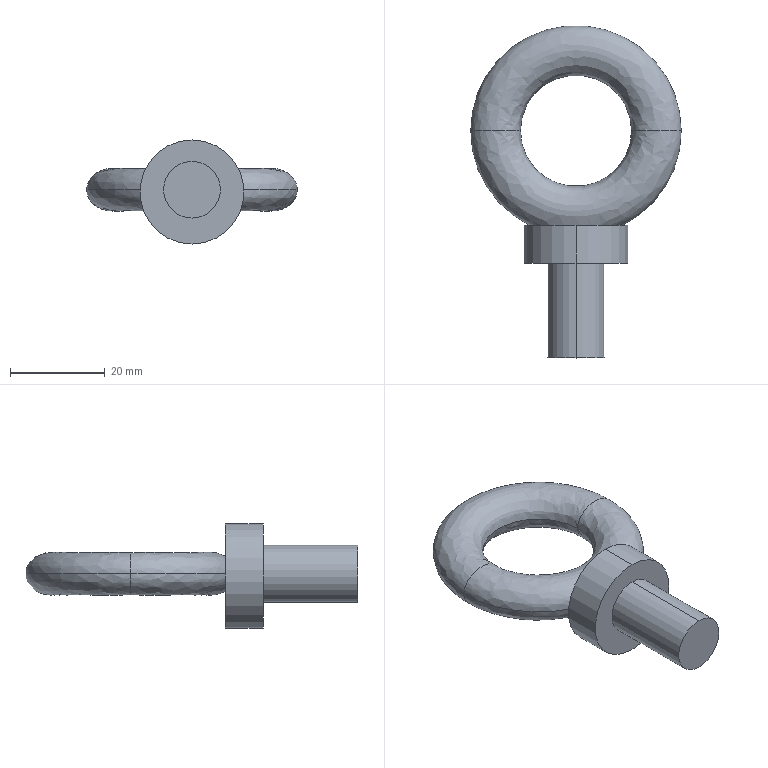Component | SolidWorks | M12LiftingEye-1 | 1 solid | 11 faces | box 44.49 x 70.25 x 22 mm | volume 13093 mm3 | spline 4 | cylinder 4 | plane 3 | commonest cylinder face diameters 12 x2 22 x2
build123d program:
from build123d import *

# Parameters (mm, degrees)
SKETCH2_RX          = 5.25
SKETCH2_RY          = 4.5
SKETCH3_R           = 11
BOSS_EXTRUDE1_DEPTH = 8
SKETCH4_R           = 6
BOSS_EXTRUDE2_DEPTH = 20


with BuildPart() as part:
    # Sweep1: sweep along a path in Sketch1
    with BuildLine(Plane.XY) as sweep1_path:
        CenterArc((0, 0), 17, 0, 360)
    # Sketch2 → Sweep1 (sweep)
    with BuildSketch(Plane(origin=(0, 0, 0), x_dir=(1, 0, 0), z_dir=(0, 1, 0))):
        with Locations(Location((16.996, 0), (0, 0, 180))):
            Ellipse(SKETCH2_RX, SKETCH2_RY)
    sweep(path=sweep1_path.line)

    # Sketch3 → Boss-Extrude1 (add)
    with BuildSketch(Plane(origin=(0, -20, 0), x_dir=(1, 0, 0), z_dir=(0, 1, 0))):
        with Locations(Location((0, 0.4774, 0), (0, 0, 270))):
            Circle(SKETCH3_R)
    extrude(amount=-BOSS_EXTRUDE1_DEPTH)

    # Sketch4 → Boss-Extrude2 (add)
    with BuildSketch(Plane.XZ.offset(28)):
        with Locations(Location((0, 0, 0), (0, 0, 90))):
            Circle(SKETCH4_R)
    extrude(amount=BOSS_EXTRUDE2_DEPTH)


solid = part.part

# Placed as in the assembly
solid = solid.moved(Location((347.082, 921.072, 1378.206), (0, 0, 0)))
STEP:
#1=COLOUR_RGB('',0.7922,0.8196,0.9333);
#2=FILL_AREA_STYLE_COLOUR('',#1);
#3=FILL_AREA_STYLE('',(#2));
#4=SURFACE_STYLE_FILL_AREA(#3);
#5=SURFACE_SIDE_STYLE('',(#4));
#6=SURFACE_STYLE_USAGE(.BOTH.,#5);
#7=PRESENTATION_STYLE_ASSIGNMENT((#6));
#8=CARTESIAN_POINT('',(14.127,36.263,54.26));
#9=VERTEX_POINT('',#8);
#10=CARTESIAN_POINT('',(13.202,36.263,54.26));
#11=VERTEX_POINT('',#10);
#12=CARTESIAN_POINT('',(13.665,36.263,54.26));
#13=DIRECTION('',(0.,0.,-1.));
#14=DIRECTION('',(1.,0.,0.));
#15=AXIS2_PLACEMENT_3D('',#12,#13,#14);
#16=CIRCLE('',#15,0.4624);
#17=EDGE_CURVE('',#9,#11,#16,.T.);
#18=ORIENTED_EDGE('',*,*,#17,.T.);
#19=CARTESIAN_POINT('',(12.789,36.263,54.26));
#20=VERTEX_POINT('',#19);
#21=CARTESIAN_POINT('',(13.202,36.263,54.26));
#22=CARTESIAN_POINT('',(13.202,36.263,54.614));
#23=CARTESIAN_POINT('',(12.789,36.263,54.614));
#24=CARTESIAN_POINT('',(12.789,36.263,54.26));
#25=(BOUNDED_CURVE()B_SPLINE_CURVE(3,(#21,#22,#23,#24),.UNSPECIFIED.,.F.,.T.)B_SPLINE_CURVE_WITH_KNOTS((4,4),(0.,3.142),.UNSPECIFIED.)CURVE()GEOMETRIC_REPRESENTATION_ITEM()RATIONAL_B_SPLINE_CURVE((1.,0.3333,0.3333,1.))REPRESENTATION_ITEM(''));
#26=EDGE_CURVE('',#11,#20,#25,.T.);
#27=ORIENTED_EDGE('',*,*,#26,.T.);
#28=CARTESIAN_POINT('',(13.281,35.475,54.26));
#29=VERTEX_POINT('',#28);
#30=CARTESIAN_POINT('',(13.665,36.263,54.26));
#31=DIRECTION('',(0.,0.,-1.));
#32=DIRECTION('',(1.,0.,0.));
#33=AXIS2_PLACEMENT_3D('',#30,#31,#32);
#34=CIRCLE('',#33,0.8758);
#35=EDGE_CURVE('',#29,#20,#34,.T.);
#36=ORIENTED_EDGE('',*,*,#35,.F.);
#37=CARTESIAN_POINT('',(14.048,35.475,54.26));
#38=VERTEX_POINT('',#37);
#39=CARTESIAN_POINT('',(13.281,35.475,54.26));
#40=CARTESIAN_POINT('',(13.281,35.475,54.265));
#41=CARTESIAN_POINT('',(13.282,35.475,54.269));
#42=CARTESIAN_POINT('',(13.284,35.475,54.278));
#43=CARTESIAN_POINT('',(13.285,35.475,54.283));
#44=CARTESIAN_POINT('',(13.29,35.475,54.296));
#45=CARTESIAN_POINT('',(13.296,35.475,54.304));
#46=CARTESIAN_POINT('',(13.307,35.475,54.318));
#47=CARTESIAN_POINT('',(13.314,35.475,54.324));
#48=CARTESIAN_POINT('',(13.329,35.475,54.336));
#49=CARTESIAN_POINT('',(13.336,35.475,54.341));
#50=CARTESIAN_POINT('',(13.36,35.475,54.355));
#51=CARTESIAN_POINT('',(13.377,35.475,54.362));
#52=CARTESIAN_POINT('',(13.412,35.475,54.375));
#53=CARTESIAN_POINT('',(13.429,35.475,54.38));
#54=CARTESIAN_POINT('',(13.483,35.475,54.392));
#55=CARTESIAN_POINT('',(13.519,35.475,54.397));
#56=CARTESIAN_POINT('',(13.574,35.475,54.402));
#57=CARTESIAN_POINT('',(13.592,35.475,54.403));
#58=CARTESIAN_POINT('',(13.629,35.475,54.405));
#59=CARTESIAN_POINT('',(13.647,35.475,54.405));
#60=CARTESIAN_POINT('',(13.702,35.475,54.405));
#61=CARTESIAN_POINT('',(13.739,35.475,54.404));
#62=CARTESIAN_POINT('',(13.811,35.475,54.397));
#63=CARTESIAN_POINT('',(13.847,35.475,54.392));
#64=CARTESIAN_POINT('',(13.901,35.475,54.38));
#65=CARTESIAN_POINT('',(13.918,35.475,54.375));
#66=CARTESIAN_POINT('',(13.953,35.475,54.362));
#67=CARTESIAN_POINT('',(13.969,35.475,54.355));
#68=CARTESIAN_POINT('',(13.993,35.475,54.341));
#69=CARTESIAN_POINT('',(14.001,35.475,54.336));
#70=CARTESIAN_POINT('',(14.015,35.475,54.324));
#71=CARTESIAN_POINT('',(14.022,35.475,54.318));
#72=CARTESIAN_POINT('',(14.034,35.475,54.304));
#73=CARTESIAN_POINT('',(14.039,35.475,54.296));
#74=CARTESIAN_POINT('',(14.046,35.475,54.279));
#75=CARTESIAN_POINT('',(14.048,35.475,54.269));
#76=CARTESIAN_POINT('',(14.048,35.475,54.26));
#77=B_SPLINE_CURVE_WITH_KNOTS('',3,(#39,#40,#41,#42,#43,#44,#45,#46,#47,#48,#49,#50,#51,#52,#53,#54,#55,#56,#57,#58,#59,#60,#61,#62,#63,#64,#65,#66,#67,#68,#69,#70,#71,#72,#73,#74,#75,#76),.UNSPECIFIED.,.F.,.F.,(4,2,2,2,2,2,2,2,2,2,2,2,2,2,2,2,2,2,4),(0.03335,0.03369,0.03404,0.03473,0.03543,0.03612,0.03751,0.03889,0.04167,0.04305,0.04444,0.04721,0.04999,0.05138,0.05276,0.05346,0.05415,0.05484,0.05554),.UNSPECIFIED.);
#78=EDGE_CURVE('',#29,#38,#77,.T.);
#79=ORIENTED_EDGE('',*,*,#78,.T.);
#80=CARTESIAN_POINT('',(14.54,36.263,54.26));
#81=VERTEX_POINT('',#80);
#82=CARTESIAN_POINT('',(13.665,36.263,54.26));
#83=DIRECTION('',(0.,0.,-1.));
#84=DIRECTION('',(1.,0.,0.));
#85=AXIS2_PLACEMENT_3D('',#82,#83,#84);
#86=CIRCLE('',#85,0.8758);
#87=EDGE_CURVE('',#81,#38,#86,.T.);
#88=ORIENTED_EDGE('',*,*,#87,.F.);
#89=CARTESIAN_POINT('',(14.127,36.263,54.26));
#90=CARTESIAN_POINT('',(14.127,36.263,54.614));
#91=CARTESIAN_POINT('',(14.54,36.263,54.614));
#92=CARTESIAN_POINT('',(14.54,36.263,54.26));
#93=(BOUNDED_CURVE()B_SPLINE_CURVE(3,(#89,#90,#91,#92),.UNSPECIFIED.,.F.,.T.)B_SPLINE_CURVE_WITH_KNOTS((4,4),(0.,3.142),.UNSPECIFIED.)CURVE()GEOMETRIC_REPRESENTATION_ITEM()RATIONAL_B_SPLINE_CURVE((1.,0.3333,0.3333,1.))REPRESENTATION_ITEM(''));
#94=EDGE_CURVE('',#9,#81,#93,.T.);
#95=ORIENTED_EDGE('',*,*,#94,.F.);
#96=EDGE_LOOP('',(#18,#27,#36,#79,#88,#95));
#97=FACE_OUTER_BOUND('',#96,.T.);
#98=CARTESIAN_POINT('',(14.127,36.263,54.26));
#99=CARTESIAN_POINT('',(14.127,35.338,54.26));
#100=CARTESIAN_POINT('',(13.202,35.338,54.26));
#101=CARTESIAN_POINT('',(13.202,36.263,54.26));
#102=CARTESIAN_POINT('',(14.127,36.263,54.614));
#103=CARTESIAN_POINT('',(14.127,35.338,54.614));
#104=CARTESIAN_POINT('',(13.202,35.338,54.614));
#105=CARTESIAN_POINT('',(13.202,36.263,54.614));
#106=CARTESIAN_POINT('',(14.54,36.263,54.614));
#107=CARTESIAN_POINT('',(14.54,34.511,54.614));
#108=CARTESIAN_POINT('',(12.789,34.511,54.614));
#109=CARTESIAN_POINT('',(12.789,36.263,54.614));
#110=CARTESIAN_POINT('',(14.54,36.263,54.26));
#111=CARTESIAN_POINT('',(14.54,34.511,54.26));
#112=CARTESIAN_POINT('',(12.789,34.511,54.26));
#113=CARTESIAN_POINT('',(12.789,36.263,54.26));
#114=(BOUNDED_SURFACE()B_SPLINE_SURFACE(3,3,((#98,#99,#100,#101),(#102,#103,#104,#105),(#106,#107,#108,#109),(#110,#111,#112,#113)),.UNSPECIFIED.,.F.,.F.,.T.)B_SPLINE_SURFACE_WITH_KNOTS((4,4),(4,4),(0.,1.),(0.,1.),.UNSPECIFIED.)GEOMETRIC_REPRESENTATION_ITEM()RATIONAL_B_SPLINE_SURFACE(((1.,0.3333,0.3333,1.),(0.3333,0.1111,0.1111,0.3333),(0.3333,0.1111,0.1111,0.3333),(1.,0.3333,0.3333,1.)))REPRESENTATION_ITEM('')SURFACE());
#115=ADVANCED_FACE('',(#97),#114,.F.);
#116=ORIENTED_EDGE('',*,*,#35,.T.);
#117=CARTESIAN_POINT('',(12.789,36.263,54.26));
#118=CARTESIAN_POINT('',(12.789,36.263,53.906));
#119=CARTESIAN_POINT('',(13.202,36.263,53.906));
#120=CARTESIAN_POINT('',(13.202,36.263,54.26));
#121=(BOUNDED_CURVE()B_SPLINE_CURVE(3,(#117,#118,#119,#120),.UNSPECIFIED.,.F.,.T.)B_SPLINE_CURVE_WITH_KNOTS((4,4),(3.142,6.283),.UNSPECIFIED.)CURVE()GEOMETRIC_REPRESENTATION_ITEM()RATIONAL_B_SPLINE_CURVE((1.,0.3333,0.3333,1.))REPRESENTATION_ITEM(''));
#122=EDGE_CURVE('',#20,#11,#121,.T.);
#123=ORIENTED_EDGE('',*,*,#122,.T.);
#124=ORIENTED_EDGE('',*,*,#17,.F.);
#125=CARTESIAN_POINT('',(14.54,36.263,54.26));
#126=CARTESIAN_POINT('',(14.54,36.263,53.906));
#127=CARTESIAN_POINT('',(14.127,36.263,53.906));
#128=CARTESIAN_POINT('',(14.127,36.263,54.26));
#129=(BOUNDED_CURVE()B_SPLINE_CURVE(3,(#125,#126,#127,#128),.UNSPECIFIED.,.F.,.T.)B_SPLINE_CURVE_WITH_KNOTS((4,4),(3.142,6.283),.UNSPECIFIED.)CURVE()GEOMETRIC_REPRESENTATION_ITEM()RATIONAL_B_SPLINE_CURVE((1.,0.3333,0.3333,1.))REPRESENTATION_ITEM(''));
#130=EDGE_CURVE('',#81,#9,#129,.T.);
#131=ORIENTED_EDGE('',*,*,#130,.F.);
#132=ORIENTED_EDGE('',*,*,#87,.T.);
#133=CARTESIAN_POINT('',(14.048,35.475,54.26));
#134=CARTESIAN_POINT('',(14.048,35.475,54.255));
#135=CARTESIAN_POINT('',(14.048,35.475,54.251));
#136=CARTESIAN_POINT('',(14.046,35.475,54.242));
#137=CARTESIAN_POINT('',(14.044,35.475,54.237));
#138=CARTESIAN_POINT('',(14.039,35.475,54.224));
#139=CARTESIAN_POINT('',(14.034,35.475,54.217));
#140=CARTESIAN_POINT('',(14.022,35.475,54.202));
#141=CARTESIAN_POINT('',(14.015,35.475,54.196));
#142=CARTESIAN_POINT('',(14.001,35.475,54.184));
#143=CARTESIAN_POINT('',(13.993,35.475,54.179));
#144=CARTESIAN_POINT('',(13.969,35.475,54.165));
#145=CARTESIAN_POINT('',(13.952,35.475,54.158));
#146=CARTESIAN_POINT('',(13.918,35.475,54.145));
#147=CARTESIAN_POINT('',(13.9,35.475,54.14));
#148=CARTESIAN_POINT('',(13.847,35.475,54.128));
#149=CARTESIAN_POINT('',(13.811,35.475,54.123));
#150=CARTESIAN_POINT('',(13.738,35.475,54.116));
#151=CARTESIAN_POINT('',(13.701,35.475,54.115));
#152=CARTESIAN_POINT('',(13.628,35.475,54.115));
#153=CARTESIAN_POINT('',(13.592,35.475,54.116));
#154=CARTESIAN_POINT('',(13.519,35.475,54.123));
#155=CARTESIAN_POINT('',(13.483,35.475,54.128));
#156=CARTESIAN_POINT('',(13.429,35.475,54.14));
#157=CARTESIAN_POINT('',(13.411,35.475,54.145));
#158=CARTESIAN_POINT('',(13.377,35.475,54.158));
#159=CARTESIAN_POINT('',(13.36,35.475,54.165));
#160=CARTESIAN_POINT('',(13.337,35.475,54.179));
#161=CARTESIAN_POINT('',(13.329,35.475,54.184));
#162=CARTESIAN_POINT('',(13.314,35.475,54.196));
#163=CARTESIAN_POINT('',(13.307,35.475,54.202));
#164=CARTESIAN_POINT('',(13.295,35.475,54.216));
#165=CARTESIAN_POINT('',(13.29,35.475,54.224));
#166=CARTESIAN_POINT('',(13.285,35.475,54.237));
#167=CARTESIAN_POINT('',(13.284,35.475,54.242));
#168=CARTESIAN_POINT('',(13.282,35.475,54.251));
#169=CARTESIAN_POINT('',(13.281,35.475,54.255));
#170=CARTESIAN_POINT('',(13.281,35.475,54.26));
#171=B_SPLINE_CURVE_WITH_KNOTS('',3,(#133,#134,#135,#136,#137,#138,#139,#140,#141,#142,#143,#144,#145,#146,#147,#148,#149,#150,#151,#152,#153,#154,#155,#156,#157,#158,#159,#160,#161,#162,#163,#164,#165,#166,#167,#168,#169,#170),.UNSPECIFIED.,.F.,.F.,(4,2,2,2,2,2,2,2,2,2,2,2,2,2,2,2,2,2,4),(0.01112,0.01147,0.01181,0.01251,0.0132,0.0139,0.01529,0.01668,0.01945,0.02223,0.02501,0.02779,0.02918,0.03057,0.03126,0.03196,0.03265,0.033,0.03335),.UNSPECIFIED.);
#172=EDGE_CURVE('',#38,#29,#171,.T.);
#173=ORIENTED_EDGE('',*,*,#172,.T.);
#174=EDGE_LOOP('',(#116,#123,#124,#131,#132,#173));
#175=FACE_OUTER_BOUND('',#174,.T.);
#176=CARTESIAN_POINT('',(14.54,36.263,54.26));
#177=CARTESIAN_POINT('',(14.54,34.511,54.26));
#178=CARTESIAN_POINT('',(12.789,34.511,54.26));
#179=CARTESIAN_POINT('',(12.789,36.263,54.26));
#180=CARTESIAN_POINT('',(14.54,36.263,53.906));
#181=CARTESIAN_POINT('',(14.54,34.511,53.906));
#182=CARTESIAN_POINT('',(12.789,34.511,53.906));
#183=CARTESIAN_POINT('',(12.789,36.263,53.906));
#184=CARTESIAN_POINT('',(14.127,36.263,53.906));
#185=CARTESIAN_POINT('',(14.127,35.338,53.906));
#186=CARTESIAN_POINT('',(13.202,35.338,53.906));
#187=CARTESIAN_POINT('',(13.202,36.263,53.906));
#188=CARTESIAN_POINT('',(14.127,36.263,54.26));
#189=CARTESIAN_POINT('',(14.127,35.338,54.26));
#190=CARTESIAN_POINT('',(13.202,35.338,54.26));
#191=CARTESIAN_POINT('',(13.202,36.263,54.26));
#192=(BOUNDED_SURFACE()B_SPLINE_SURFACE(3,3,((#176,#177,#178,#179),(#180,#181,#182,#183),(#184,#185,#186,#187),(#188,#189,#190,#191)),.UNSPECIFIED.,.F.,.F.,.F.)B_SPLINE_SURFACE_WITH_KNOTS((4,4),(4,4),(0.,1.),(0.,1.),.UNSPECIFIED.)GEOMETRIC_REPRESENTATION_ITEM()RATIONAL_B_SPLINE_SURFACE(((1.,0.3333,0.3333,1.),(0.3333,0.1111,0.1111,0.3333),(0.3333,0.1111,0.1111,0.3333),(1.,0.3333,0.3333,1.)))REPRESENTATION_ITEM('')SURFACE());
#193=ADVANCED_FACE('',(#175),#192,.F.);
#194=CARTESIAN_POINT('',(13.665,34.373,54.024));
#195=VERTEX_POINT('',#194);
#196=CARTESIAN_POINT('',(13.665,34.373,54.496));
#197=VERTEX_POINT('',#196);
#198=CARTESIAN_POINT('',(13.665,34.373,54.26));
#199=DIRECTION('',(0.,-1.,0.));
#200=DIRECTION('',(0.,0.,-1.));
#201=AXIS2_PLACEMENT_3D('',#198,#199,#200);
#202=CIRCLE('',#201,0.2362);
#203=EDGE_CURVE('',#195,#197,#202,.T.);
#204=ORIENTED_EDGE('',*,*,#203,.F.);
#205=CARTESIAN_POINT('',(13.665,35.16,54.024));
#206=VERTEX_POINT('',#205);
#207=CARTESIAN_POINT('',(13.665,34.373,54.024));
#208=DIRECTION('',(0.,1.,0.));
#209=VECTOR('',#208,39.37);
#210=LINE('',#207,#209);
#211=EDGE_CURVE('',#195,#206,#210,.T.);
#212=ORIENTED_EDGE('',*,*,#211,.T.);
#213=CARTESIAN_POINT('',(13.665,35.16,54.496));
#214=VERTEX_POINT('',#213);
#215=CARTESIAN_POINT('',(13.665,35.16,54.26));
#216=DIRECTION('',(0.,-1.,0.));
#217=DIRECTION('',(0.,0.,1.));
#218=AXIS2_PLACEMENT_3D('',#215,#216,#217);
#219=CIRCLE('',#218,0.2362);
#220=EDGE_CURVE('',#206,#214,#219,.T.);
#221=ORIENTED_EDGE('',*,*,#220,.T.);
#222=CARTESIAN_POINT('',(13.665,34.373,54.496));
#223=DIRECTION('',(0.,1.,0.));
#224=VECTOR('',#223,39.37);
#225=LINE('',#222,#224);
#226=EDGE_CURVE('',#197,#214,#225,.T.);
#227=ORIENTED_EDGE('',*,*,#226,.F.);
#228=EDGE_LOOP('',(#204,#212,#221,#227));
#229=FACE_OUTER_BOUND('',#228,.T.);
#230=CARTESIAN_POINT('',(13.665,34.373,54.26));
#231=DIRECTION('',(0.,1.,0.));
#232=DIRECTION('',(0.,0.,1.));
#233=AXIS2_PLACEMENT_3D('',#230,#231,#232);
#234=CYLINDRICAL_SURFACE('',#233,0.2362);
#235=ADVANCED_FACE('',(#229),#234,.T.);
#236=ORIENTED_EDGE('',*,*,#122,.F.);
#237=CARTESIAN_POINT('',(13.665,36.263,54.26));
#238=DIRECTION('',(0.,0.,-1.));
#239=DIRECTION('',(1.,0.,0.));
#240=AXIS2_PLACEMENT_3D('',#237,#238,#239);
#241=CIRCLE('',#240,0.8758);
#242=EDGE_CURVE('',#20,#81,#241,.T.);
#243=ORIENTED_EDGE('',*,*,#242,.T.);
#244=ORIENTED_EDGE('',*,*,#130,.T.);
#245=CARTESIAN_POINT('',(13.665,36.263,54.26));
#246=DIRECTION('',(0.,0.,-1.));
#247=DIRECTION('',(1.,0.,0.));
#248=AXIS2_PLACEMENT_3D('',#245,#246,#247);
#249=CIRCLE('',#248,0.4624);
#250=EDGE_CURVE('',#11,#9,#249,.T.);
#251=ORIENTED_EDGE('',*,*,#250,.F.);
#252=EDGE_LOOP('',(#236,#243,#244,#251));
#253=FACE_OUTER_BOUND('',#252,.T.);
#254=CARTESIAN_POINT('',(12.789,36.263,54.26));
#255=CARTESIAN_POINT('',(12.789,38.014,54.26));
#256=CARTESIAN_POINT('',(14.54,38.014,54.26));
#257=CARTESIAN_POINT('',(14.54,36.263,54.26));
#258=CARTESIAN_POINT('',(12.789,36.263,53.906));
#259=CARTESIAN_POINT('',(12.789,38.014,53.906));
#260=CARTESIAN_POINT('',(14.54,38.014,53.906));
#261=CARTESIAN_POINT('',(14.54,36.263,53.906));
#262=CARTESIAN_POINT('',(13.202,36.263,53.906));
#263=CARTESIAN_POINT('',(13.202,37.188,53.906));
#264=CARTESIAN_POINT('',(14.127,37.188,53.906));
#265=CARTESIAN_POINT('',(14.127,36.263,53.906));
#266=CARTESIAN_POINT('',(13.202,36.263,54.26));
#267=CARTESIAN_POINT('',(13.202,37.188,54.26));
#268=CARTESIAN_POINT('',(14.127,37.188,54.26));
#269=CARTESIAN_POINT('',(14.127,36.263,54.26));
#270=(BOUNDED_SURFACE()B_SPLINE_SURFACE(3,3,((#254,#255,#256,#257),(#258,#259,#260,#261),(#262,#263,#264,#265),(#266,#267,#268,#269)),.UNSPECIFIED.,.F.,.F.,.T.)B_SPLINE_SURFACE_WITH_KNOTS((4,4),(4,4),(0.,1.),(0.,1.),.UNSPECIFIED.)GEOMETRIC_REPRESENTATION_ITEM()RATIONAL_B_SPLINE_SURFACE(((1.,0.3333,0.3333,1.),(0.3333,0.1111,0.1111,0.3333),(0.3333,0.1111,0.1111,0.3333),(1.,0.3333,0.3333,1.)))REPRESENTATION_ITEM('')SURFACE());
#271=ADVANCED_FACE('',(#253),#270,.F.);
#272=CARTESIAN_POINT('',(13.665,35.16,54.674));
#273=VERTEX_POINT('',#272);
#274=CARTESIAN_POINT('',(13.665,35.16,53.808));
#275=VERTEX_POINT('',#274);
#276=CARTESIAN_POINT('',(13.665,35.16,54.241));
#277=DIRECTION('',(0.,1.,0.));
#278=DIRECTION('',(0.,0.,1.));
#279=AXIS2_PLACEMENT_3D('',#276,#277,#278);
#280=CIRCLE('',#279,0.4331);
#281=EDGE_CURVE('',#273,#275,#280,.T.);
#282=ORIENTED_EDGE('',*,*,#281,.T.);
#283=CARTESIAN_POINT('',(13.665,35.475,53.808));
#284=VERTEX_POINT('',#283);
#285=CARTESIAN_POINT('',(13.665,35.16,53.808));
#286=DIRECTION('',(0.,1.,0.));
#287=VECTOR('',#286,39.37);
#288=LINE('',#285,#287);
#289=EDGE_CURVE('',#275,#284,#288,.T.);
#290=ORIENTED_EDGE('',*,*,#289,.T.);
#291=CARTESIAN_POINT('',(13.665,35.475,54.674));
#292=VERTEX_POINT('',#291);
#293=CARTESIAN_POINT('',(13.665,35.475,54.241));
#294=DIRECTION('',(0.,1.,0.));
#295=DIRECTION('',(0.,0.,1.));
#296=AXIS2_PLACEMENT_3D('',#293,#294,#295);
#297=CIRCLE('',#296,0.4331);
#298=EDGE_CURVE('',#292,#284,#297,.T.);
#299=ORIENTED_EDGE('',*,*,#298,.F.);
#300=CARTESIAN_POINT('',(13.665,35.16,54.674));
#301=DIRECTION('',(0.,1.,0.));
#302=VECTOR('',#301,39.37);
#303=LINE('',#300,#302);
#304=EDGE_CURVE('',#273,#292,#303,.T.);
#305=ORIENTED_EDGE('',*,*,#304,.F.);
#306=EDGE_LOOP('',(#282,#290,#299,#305));
#307=FACE_OUTER_BOUND('',#306,.T.);
#308=CARTESIAN_POINT('',(13.665,35.16,54.241));
#309=DIRECTION('',(0.,1.,0.));
#310=DIRECTION('',(0.,0.,1.));
#311=AXIS2_PLACEMENT_3D('',#308,#309,#310);
#312=CYLINDRICAL_SURFACE('',#311,0.4331);
#313=ADVANCED_FACE('',(#307),#312,.T.);
#314=ORIENTED_EDGE('',*,*,#281,.F.);
#315=CARTESIAN_POINT('',(13.665,35.16,54.241));
#316=DIRECTION('',(0.,1.,0.));
#317=DIRECTION('',(0.,0.,1.));
#318=AXIS2_PLACEMENT_3D('',#315,#316,#317);
#319=CIRCLE('',#318,0.4331);
#320=EDGE_CURVE('',#275,#273,#319,.T.);
#321=ORIENTED_EDGE('',*,*,#320,.F.);
#322=EDGE_LOOP('',(#314,#321));
#323=FACE_OUTER_BOUND('',#322,.T.);
#324=CARTESIAN_POINT('',(13.665,35.16,54.26));
#325=DIRECTION('',(0.,-1.,0.));
#326=DIRECTION('',(0.,0.,1.));
#327=AXIS2_PLACEMENT_3D('',#324,#325,#326);
#328=CIRCLE('',#327,0.2362);
#329=EDGE_CURVE('',#214,#206,#328,.T.);
#330=ORIENTED_EDGE('',*,*,#329,.F.);
#331=ORIENTED_EDGE('',*,*,#220,.F.);
#332=EDGE_LOOP('',(#330,#331));
#333=FACE_BOUND('',#332,.T.);
#334=CARTESIAN_POINT('',(13.665,35.16,54.241));
#335=DIRECTION('',(0.,1.,0.));
#336=DIRECTION('',(0.,0.,1.));
#337=AXIS2_PLACEMENT_3D('',#334,#335,#336);
#338=PLANE('',#337);
#339=ADVANCED_FACE('',(#323,#333),#338,.F.);
#340=ORIENTED_EDGE('',*,*,#298,.T.);
#341=CARTESIAN_POINT('',(13.665,35.475,54.241));
#342=DIRECTION('',(0.,1.,0.));
#343=DIRECTION('',(0.,0.,1.));
#344=AXIS2_PLACEMENT_3D('',#341,#342,#343);
#345=CIRCLE('',#344,0.4331);
#346=EDGE_CURVE('',#284,#292,#345,.T.);
#347=ORIENTED_EDGE('',*,*,#346,.T.);
#348=EDGE_LOOP('',(#340,#347));
#349=FACE_OUTER_BOUND('',#348,.T.);
#350=ORIENTED_EDGE('',*,*,#172,.F.);
#351=ORIENTED_EDGE('',*,*,#78,.F.);
#352=EDGE_LOOP('',(#350,#351));
#353=FACE_BOUND('',#352,.T.);
#354=CARTESIAN_POINT('',(13.665,35.475,54.241));
#355=DIRECTION('',(0.,1.,0.));
#356=DIRECTION('',(0.,0.,1.));
#357=AXIS2_PLACEMENT_3D('',#354,#355,#356);
#358=PLANE('',#357);
#359=ADVANCED_FACE('',(#349,#353),#358,.T.);
#360=ORIENTED_EDGE('',*,*,#289,.F.);
#361=ORIENTED_EDGE('',*,*,#320,.T.);
#362=ORIENTED_EDGE('',*,*,#304,.T.);
#363=ORIENTED_EDGE('',*,*,#346,.F.);
#364=EDGE_LOOP('',(#360,#361,#362,#363));
#365=FACE_OUTER_BOUND('',#364,.T.);
#366=CARTESIAN_POINT('',(13.665,35.16,54.241));
#367=DIRECTION('',(0.,1.,0.));
#368=DIRECTION('',(0.,0.,1.));
#369=AXIS2_PLACEMENT_3D('',#366,#367,#368);
#370=CYLINDRICAL_SURFACE('',#369,0.4331);
#371=ADVANCED_FACE('',(#365),#370,.T.);
#372=ORIENTED_EDGE('',*,*,#26,.F.);
#373=ORIENTED_EDGE('',*,*,#250,.T.);
#374=ORIENTED_EDGE('',*,*,#94,.T.);
#375=ORIENTED_EDGE('',*,*,#242,.F.);
#376=EDGE_LOOP('',(#372,#373,#374,#375));
#377=FACE_OUTER_BOUND('',#376,.T.);
#378=CARTESIAN_POINT('',(13.202,36.263,54.26));
#379=CARTESIAN_POINT('',(13.202,37.188,54.26));
#380=CARTESIAN_POINT('',(14.127,37.188,54.26));
#381=CARTESIAN_POINT('',(14.127,36.263,54.26));
#382=CARTESIAN_POINT('',(13.202,36.263,54.614));
#383=CARTESIAN_POINT('',(13.202,37.188,54.614));
#384=CARTESIAN_POINT('',(14.127,37.188,54.614));
#385=CARTESIAN_POINT('',(14.127,36.263,54.614));
#386=CARTESIAN_POINT('',(12.789,36.263,54.614));
#387=CARTESIAN_POINT('',(12.789,38.014,54.614));
#388=CARTESIAN_POINT('',(14.54,38.014,54.614));
#389=CARTESIAN_POINT('',(14.54,36.263,54.614));
#390=CARTESIAN_POINT('',(12.789,36.263,54.26));
#391=CARTESIAN_POINT('',(12.789,38.014,54.26));
#392=CARTESIAN_POINT('',(14.54,38.014,54.26));
#393=CARTESIAN_POINT('',(14.54,36.263,54.26));
#394=(BOUNDED_SURFACE()B_SPLINE_SURFACE(3,3,((#378,#379,#380,#381),(#382,#383,#384,#385),(#386,#387,#388,#389),(#390,#391,#392,#393)),.UNSPECIFIED.,.F.,.F.,.F.)B_SPLINE_SURFACE_WITH_KNOTS((4,4),(4,4),(0.,1.),(0.,1.),.UNSPECIFIED.)GEOMETRIC_REPRESENTATION_ITEM()RATIONAL_B_SPLINE_SURFACE(((1.,0.3333,0.3333,1.),(0.3333,0.1111,0.1111,0.3333),(0.3333,0.1111,0.1111,0.3333),(1.,0.3333,0.3333,1.)))REPRESENTATION_ITEM('')SURFACE());
#395=ADVANCED_FACE('',(#377),#394,.F.);
#396=ORIENTED_EDGE('',*,*,#211,.F.);
#397=CARTESIAN_POINT('',(13.665,34.373,54.26));
#398=DIRECTION('',(0.,-1.,0.));
#399=DIRECTION('',(0.,0.,-1.));
#400=AXIS2_PLACEMENT_3D('',#397,#398,#399);
#401=CIRCLE('',#400,0.2362);
#402=EDGE_CURVE('',#197,#195,#401,.T.);
#403=ORIENTED_EDGE('',*,*,#402,.F.);
#404=ORIENTED_EDGE('',*,*,#226,.T.);
#405=ORIENTED_EDGE('',*,*,#329,.T.);
#406=EDGE_LOOP('',(#396,#403,#404,#405));
#407=FACE_OUTER_BOUND('',#406,.T.);
#408=CARTESIAN_POINT('',(13.665,34.373,54.26));
#409=DIRECTION('',(0.,1.,0.));
#410=DIRECTION('',(0.,0.,1.));
#411=AXIS2_PLACEMENT_3D('',#408,#409,#410);
#412=CYLINDRICAL_SURFACE('',#411,0.2362);
#413=ADVANCED_FACE('',(#407),#412,.T.);
#414=ORIENTED_EDGE('',*,*,#402,.T.);
#415=ORIENTED_EDGE('',*,*,#203,.T.);
#416=EDGE_LOOP('',(#414,#415));
#417=FACE_OUTER_BOUND('',#416,.T.);
#418=CARTESIAN_POINT('',(13.665,34.373,54.26));
#419=DIRECTION('',(0.,-1.,0.));
#420=DIRECTION('',(0.,0.,-1.));
#421=AXIS2_PLACEMENT_3D('',#418,#419,#420);
#422=PLANE('',#421);
#423=ADVANCED_FACE('',(#417),#422,.T.);
#424=CLOSED_SHELL('',(#115,#193,#235,#271,#313,#339,#359,#371,#395,#413,#423));
#425=MANIFOLD_SOLID_BREP('',#424);
#426=STYLED_ITEM('',(#7),#425);
#427=(LENGTH_UNIT()NAMED_UNIT(*)SI_UNIT($,.METRE.));
#428=LENGTH_MEASURE_WITH_UNIT(LENGTH_MEASURE(0.0254),#427);
#429=DIMENSIONAL_EXPONENTS(1.,0.,0.,0.,0.,0.,0.);
#430=(CONVERSION_BASED_UNIT('',#428)LENGTH_UNIT()NAMED_UNIT(#429));
#431=UNCERTAINTY_MEASURE_WITH_UNIT(LENGTH_MEASURE(0.00001),#430,'','');
#432=(NAMED_UNIT(*)PLANE_ANGLE_UNIT()SI_UNIT($,.RADIAN.));
#433=(NAMED_UNIT(*)SI_UNIT($,.STERADIAN.)SOLID_ANGLE_UNIT());
#434=(GEOMETRIC_REPRESENTATION_CONTEXT(3)GLOBAL_UNCERTAINTY_ASSIGNED_CONTEXT((#431))GLOBAL_UNIT_ASSIGNED_CONTEXT((#430,#432,#433))REPRESENTATION_CONTEXT('',''));
#435=MECHANICAL_DESIGN_GEOMETRIC_PRESENTATION_REPRESENTATION('',(#426),#434);
#436=CARTESIAN_POINT('',(0.,0.,0.));
#437=DIRECTION('',(0.,0.,1.));
#438=DIRECTION('',(1.,0.,0.));
#439=AXIS2_PLACEMENT_3D('',#436,#437,#438);
#440=(LENGTH_UNIT()NAMED_UNIT(*)SI_UNIT($,.METRE.));
#441=LENGTH_MEASURE_WITH_UNIT(LENGTH_MEASURE(0.0254),#440);
#442=DIMENSIONAL_EXPONENTS(1.,0.,0.,0.,0.,0.,0.);
#443=(CONVERSION_BASED_UNIT('',#441)LENGTH_UNIT()NAMED_UNIT(#442));
#444=UNCERTAINTY_MEASURE_WITH_UNIT(LENGTH_MEASURE(0.00001),#443,'','');
#445=(NAMED_UNIT(*)PLANE_ANGLE_UNIT()SI_UNIT($,.RADIAN.));
#446=(NAMED_UNIT(*)SI_UNIT($,.STERADIAN.)SOLID_ANGLE_UNIT());
#447=(GEOMETRIC_REPRESENTATION_CONTEXT(3)GLOBAL_UNCERTAINTY_ASSIGNED_CONTEXT((#444))GLOBAL_UNIT_ASSIGNED_CONTEXT((#443,#445,#446))REPRESENTATION_CONTEXT('',''));
#448=ADVANCED_BREP_SHAPE_REPRESENTATION('',(#425,#439),#447);
#449=PRESENTATION_LAYER_ASSIGNMENT('','',(#426));